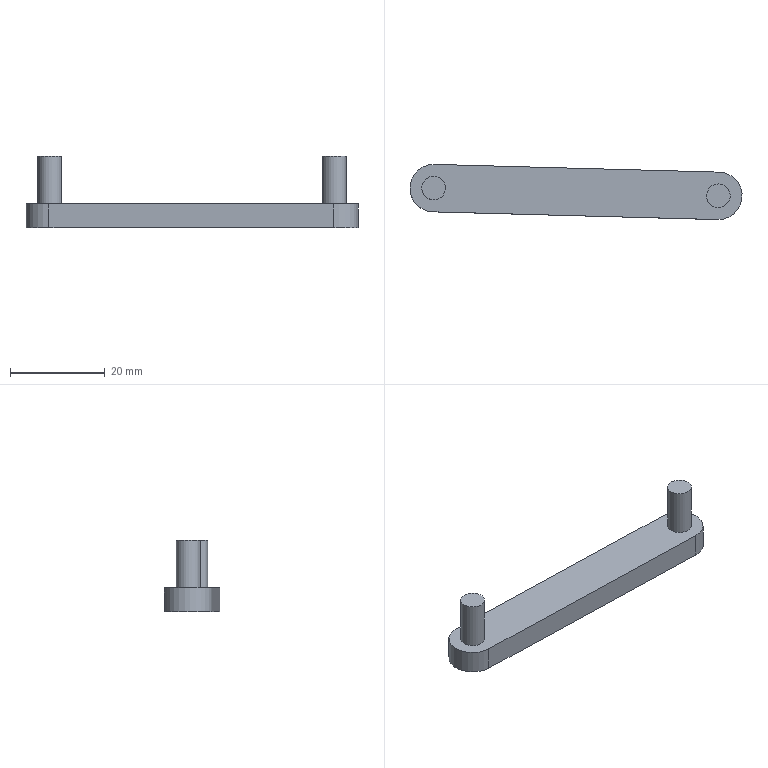Component | NX | CONN_ROD_2 | 1 solid | 10 faces | box 69.98 x 11.63 x 15 mm | volume 3785 mm3 | plane 6 | cylinder 4 | commonest cylinder face diameters 10 x2 5 x2
STEP:
#1=CARTESIAN_POINT('',(0.,0.,0.));
#2=DIRECTION('',(0.,0.,1.));
#3=DIRECTION('',(1.,0.,0.));
#4=AXIS2_PLACEMENT_3D('',#1,#2,#3);
#5=CARTESIAN_POINT('',(-59.864,-73.595,-2.5));
#6=VERTEX_POINT('',#5);
#7=CARTESIAN_POINT('',(-119.842,-71.969,-2.5));
#8=VERTEX_POINT('',#7);
#9=CARTESIAN_POINT('',(-59.864,-73.595,-2.5));
#10=DIRECTION('',(-0.9996,0.0271,0.));
#11=VECTOR('',#10,1.);
#12=LINE('',#9,#11);
#13=CARTESIAN_POINT('',(-59.864,-73.595,2.5));
#14=DIRECTION('',(-0.0271,-0.9996,0.));
#15=DIRECTION('',(0.9996,-0.0271,0.));
#16=AXIS2_PLACEMENT_3D('',#13,#14,#15);
#17=PLANE('',#16);
#18=CARTESIAN_POINT('',(0.,-5.));
#19=DIRECTION('',(-1.,0.));
#20=VECTOR('',#19,1.);
#21=LINE('',#18,#20);
#22=(GEOMETRIC_REPRESENTATION_CONTEXT(2)PARAMETRIC_REPRESENTATION_CONTEXT()REPRESENTATION_CONTEXT('',''));
#23=DEFINITIONAL_REPRESENTATION('',(#21),#22);
#24=PCURVE('',#17,#23);
#25=CARTESIAN_POINT('',(-119.978,-76.967,-2.5));
#26=DIRECTION('',(0.,0.,1.));
#27=DIRECTION('',(-0.0271,-0.9996,0.));
#28=AXIS2_PLACEMENT_3D('',#25,#26,#27);
#29=PLANE('',#28);
#30=CARTESIAN_POINT('',(-5.,60.));
#31=DIRECTION('',(-0.,-1.));
#32=VECTOR('',#31,1.);
#33=LINE('',#30,#32);
#34=(GEOMETRIC_REPRESENTATION_CONTEXT(2)PARAMETRIC_REPRESENTATION_CONTEXT()REPRESENTATION_CONTEXT('',''));
#35=DEFINITIONAL_REPRESENTATION('',(#33),#34);
#36=PCURVE('',#29,#35);
#37=SURFACE_CURVE('',#12,(#24,#36),.PCURVE_S1.);
#38=EDGE_CURVE('',#6,#8,#37,.T.);
#39=ORIENTED_EDGE('',*,*,#38,.T.);
#40=CARTESIAN_POINT('',(-119.842,-71.969,2.5));
#41=VERTEX_POINT('',#40);
#42=CARTESIAN_POINT('',(-119.842,-71.969,2.5));
#43=DIRECTION('',(0.,0.,-1.));
#44=VECTOR('',#43,1.);
#45=LINE('',#42,#44);
#46=CARTESIAN_POINT('',(-60.,0.));
#47=DIRECTION('',(0.,-1.));
#48=VECTOR('',#47,1.);
#49=LINE('',#46,#48);
#50=(GEOMETRIC_REPRESENTATION_CONTEXT(2)PARAMETRIC_REPRESENTATION_CONTEXT()REPRESENTATION_CONTEXT('',''));
#51=DEFINITIONAL_REPRESENTATION('',(#49),#50);
#52=PCURVE('',#17,#51);
#53=CARTESIAN_POINT('',(-119.978,-76.967,2.5));
#54=DIRECTION('',(0.,0.,-1.));
#55=DIRECTION('',(0.0271,0.9996,0.));
#56=AXIS2_PLACEMENT_3D('',#53,#54,#55);
#57=CYLINDRICAL_SURFACE('',#56,5.);
#58=CARTESIAN_POINT('',(6.283,0.));
#59=DIRECTION('',(0.,1.));
#60=VECTOR('',#59,1.);
#61=LINE('',#58,#60);
#62=(GEOMETRIC_REPRESENTATION_CONTEXT(2)PARAMETRIC_REPRESENTATION_CONTEXT()REPRESENTATION_CONTEXT('',''));
#63=DEFINITIONAL_REPRESENTATION('',(#61),#62);
#64=PCURVE('',#57,#63);
#65=SURFACE_CURVE('',#45,(#52,#64),.PCURVE_S1.);
#66=EDGE_CURVE('',#41,#8,#65,.T.);
#67=ORIENTED_EDGE('',*,*,#66,.F.);
#68=CARTESIAN_POINT('',(-59.864,-73.595,2.5));
#69=VERTEX_POINT('',#68);
#70=CARTESIAN_POINT('',(-59.864,-73.595,2.5));
#71=DIRECTION('',(-0.9996,0.0271,0.));
#72=VECTOR('',#71,1.);
#73=LINE('',#70,#72);
#74=CARTESIAN_POINT('',(0.,0.));
#75=DIRECTION('',(-1.,0.));
#76=VECTOR('',#75,1.);
#77=LINE('',#74,#76);
#78=(GEOMETRIC_REPRESENTATION_CONTEXT(2)PARAMETRIC_REPRESENTATION_CONTEXT()REPRESENTATION_CONTEXT('',''));
#79=DEFINITIONAL_REPRESENTATION('',(#77),#78);
#80=PCURVE('',#17,#79);
#81=CARTESIAN_POINT('',(-119.978,-76.967,2.5));
#82=DIRECTION('',(0.,0.,1.));
#83=DIRECTION('',(-0.0271,-0.9996,0.));
#84=AXIS2_PLACEMENT_3D('',#81,#82,#83);
#85=PLANE('',#84);
#86=CARTESIAN_POINT('',(-5.,60.));
#87=DIRECTION('',(-0.,-1.));
#88=VECTOR('',#87,1.);
#89=LINE('',#86,#88);
#90=(GEOMETRIC_REPRESENTATION_CONTEXT(2)PARAMETRIC_REPRESENTATION_CONTEXT()REPRESENTATION_CONTEXT('',''));
#91=DEFINITIONAL_REPRESENTATION('',(#89),#90);
#92=PCURVE('',#85,#91);
#93=SURFACE_CURVE('',#73,(#80,#92),.PCURVE_S1.);
#94=EDGE_CURVE('',#69,#41,#93,.T.);
#95=ORIENTED_EDGE('',*,*,#94,.F.);
#96=CARTESIAN_POINT('',(-59.864,-73.595,2.5));
#97=DIRECTION('',(0.,0.,-1.));
#98=VECTOR('',#97,1.);
#99=LINE('',#96,#98);
#100=CARTESIAN_POINT('',(0.,0.));
#101=DIRECTION('',(0.,-1.));
#102=VECTOR('',#101,1.);
#103=LINE('',#100,#102);
#104=(GEOMETRIC_REPRESENTATION_CONTEXT(2)PARAMETRIC_REPRESENTATION_CONTEXT()REPRESENTATION_CONTEXT('',''));
#105=DEFINITIONAL_REPRESENTATION('',(#103),#104);
#106=PCURVE('',#17,#105);
#107=CARTESIAN_POINT('',(-60.,-78.593,2.5));
#108=DIRECTION('',(0.,0.,-1.));
#109=DIRECTION('',(0.0271,0.9996,0.));
#110=AXIS2_PLACEMENT_3D('',#107,#108,#109);
#111=CYLINDRICAL_SURFACE('',#110,5.);
#112=CARTESIAN_POINT('',(0.,0.));
#113=DIRECTION('',(0.,1.));
#114=VECTOR('',#113,1.);
#115=LINE('',#112,#114);
#116=(GEOMETRIC_REPRESENTATION_CONTEXT(2)PARAMETRIC_REPRESENTATION_CONTEXT()REPRESENTATION_CONTEXT('',''));
#117=DEFINITIONAL_REPRESENTATION('',(#115),#116);
#118=PCURVE('',#111,#117);
#119=SURFACE_CURVE('',#99,(#106,#118),.PCURVE_S1.);
#120=EDGE_CURVE('',#69,#6,#119,.T.);
#121=ORIENTED_EDGE('',*,*,#120,.T.);
#122=EDGE_LOOP('',(#39,#67,#95,#121));
#123=FACE_BOUND('',#122,.T.);
#124=ADVANCED_FACE('',(#123),#17,.F.);
#125=CARTESIAN_POINT('',(-120.113,-81.965,-2.5));
#126=VERTEX_POINT('',#125);
#127=CARTESIAN_POINT('',(-119.978,-76.967,-2.5));
#128=DIRECTION('',(0.,0.,1.));
#129=DIRECTION('',(-0.0271,-0.9996,0.));
#130=AXIS2_PLACEMENT_3D('',#127,#128,#129);
#131=CIRCLE('',#130,5.);
#132=CARTESIAN_POINT('',(9.425,5.));
#133=DIRECTION('',(-1.,0.));
#134=VECTOR('',#133,1.);
#135=LINE('',#132,#134);
#136=(GEOMETRIC_REPRESENTATION_CONTEXT(2)PARAMETRIC_REPRESENTATION_CONTEXT()REPRESENTATION_CONTEXT('',''));
#137=DEFINITIONAL_REPRESENTATION('',(#135),#136);
#138=PCURVE('',#57,#137);
#139=CARTESIAN_POINT('',(0.,0.));
#140=DIRECTION('',(1.,-0.));
#141=AXIS2_PLACEMENT_2D('',#139,#140);
#142=CIRCLE('',#141,5.);
#143=(GEOMETRIC_REPRESENTATION_CONTEXT(2)PARAMETRIC_REPRESENTATION_CONTEXT()REPRESENTATION_CONTEXT('',''));
#144=DEFINITIONAL_REPRESENTATION('',(#142),#143);
#145=PCURVE('',#29,#144);
#146=SURFACE_CURVE('',#131,(#138,#145),.PCURVE_S1.);
#147=EDGE_CURVE('',#8,#126,#146,.T.);
#148=ORIENTED_EDGE('',*,*,#147,.T.);
#149=CARTESIAN_POINT('',(-120.113,-81.965,2.5));
#150=VERTEX_POINT('',#149);
#151=CARTESIAN_POINT('',(-120.113,-81.965,2.5));
#152=DIRECTION('',(0.,0.,-1.));
#153=VECTOR('',#152,1.);
#154=LINE('',#151,#153);
#155=CARTESIAN_POINT('',(3.142,0.));
#156=DIRECTION('',(0.,1.));
#157=VECTOR('',#156,1.);
#158=LINE('',#155,#157);
#159=(GEOMETRIC_REPRESENTATION_CONTEXT(2)PARAMETRIC_REPRESENTATION_CONTEXT()REPRESENTATION_CONTEXT('',''));
#160=DEFINITIONAL_REPRESENTATION('',(#158),#159);
#161=PCURVE('',#57,#160);
#162=CARTESIAN_POINT('',(-120.113,-81.965,2.5));
#163=DIRECTION('',(0.0271,0.9996,0.));
#164=DIRECTION('',(-0.9996,0.0271,0.));
#165=AXIS2_PLACEMENT_3D('',#162,#163,#164);
#166=PLANE('',#165);
#167=CARTESIAN_POINT('',(0.,0.));
#168=DIRECTION('',(0.,-1.));
#169=VECTOR('',#168,1.);
#170=LINE('',#167,#169);
#171=(GEOMETRIC_REPRESENTATION_CONTEXT(2)PARAMETRIC_REPRESENTATION_CONTEXT()REPRESENTATION_CONTEXT('',''));
#172=DEFINITIONAL_REPRESENTATION('',(#170),#171);
#173=PCURVE('',#166,#172);
#174=SURFACE_CURVE('',#154,(#161,#173),.PCURVE_S1.);
#175=EDGE_CURVE('',#150,#126,#174,.T.);
#176=ORIENTED_EDGE('',*,*,#175,.F.);
#177=CARTESIAN_POINT('',(-119.978,-76.967,2.5));
#178=DIRECTION('',(0.,0.,1.));
#179=DIRECTION('',(-0.0271,-0.9996,0.));
#180=AXIS2_PLACEMENT_3D('',#177,#178,#179);
#181=CIRCLE('',#180,5.);
#182=CARTESIAN_POINT('',(9.425,0.));
#183=DIRECTION('',(-1.,0.));
#184=VECTOR('',#183,1.);
#185=LINE('',#182,#184);
#186=(GEOMETRIC_REPRESENTATION_CONTEXT(2)PARAMETRIC_REPRESENTATION_CONTEXT()REPRESENTATION_CONTEXT('',''));
#187=DEFINITIONAL_REPRESENTATION('',(#185),#186);
#188=PCURVE('',#57,#187);
#189=CARTESIAN_POINT('',(0.,0.));
#190=DIRECTION('',(1.,-0.));
#191=AXIS2_PLACEMENT_2D('',#189,#190);
#192=CIRCLE('',#191,5.);
#193=(GEOMETRIC_REPRESENTATION_CONTEXT(2)PARAMETRIC_REPRESENTATION_CONTEXT()REPRESENTATION_CONTEXT('',''));
#194=DEFINITIONAL_REPRESENTATION('',(#192),#193);
#195=PCURVE('',#85,#194);
#196=SURFACE_CURVE('',#181,(#188,#195),.PCURVE_S1.);
#197=EDGE_CURVE('',#41,#150,#196,.T.);
#198=ORIENTED_EDGE('',*,*,#197,.F.);
#199=ORIENTED_EDGE('',*,*,#66,.T.);
#200=EDGE_LOOP('',(#148,#176,#198,#199));
#201=FACE_BOUND('',#200,.T.);
#202=ADVANCED_FACE('',(#201),#57,.T.);
#203=CARTESIAN_POINT('',(-60.136,-83.592,-2.5));
#204=VERTEX_POINT('',#203);
#205=CARTESIAN_POINT('',(-120.113,-81.965,-2.5));
#206=DIRECTION('',(0.9996,-0.0271,0.));
#207=VECTOR('',#206,1.);
#208=LINE('',#205,#207);
#209=CARTESIAN_POINT('',(0.,-5.));
#210=DIRECTION('',(-1.,0.));
#211=VECTOR('',#210,1.);
#212=LINE('',#209,#211);
#213=(GEOMETRIC_REPRESENTATION_CONTEXT(2)PARAMETRIC_REPRESENTATION_CONTEXT()REPRESENTATION_CONTEXT('',''));
#214=DEFINITIONAL_REPRESENTATION('',(#212),#213);
#215=PCURVE('',#166,#214);
#216=CARTESIAN_POINT('',(5.,0.));
#217=DIRECTION('',(0.,1.));
#218=VECTOR('',#217,1.);
#219=LINE('',#216,#218);
#220=(GEOMETRIC_REPRESENTATION_CONTEXT(2)PARAMETRIC_REPRESENTATION_CONTEXT()REPRESENTATION_CONTEXT('',''));
#221=DEFINITIONAL_REPRESENTATION('',(#219),#220);
#222=PCURVE('',#29,#221);
#223=SURFACE_CURVE('',#208,(#215,#222),.PCURVE_S1.);
#224=EDGE_CURVE('',#126,#204,#223,.T.);
#225=ORIENTED_EDGE('',*,*,#224,.T.);
#226=CARTESIAN_POINT('',(-60.136,-83.592,2.5));
#227=VERTEX_POINT('',#226);
#228=CARTESIAN_POINT('',(-60.136,-83.592,2.5));
#229=DIRECTION('',(0.,0.,-1.));
#230=VECTOR('',#229,1.);
#231=LINE('',#228,#230);
#232=CARTESIAN_POINT('',(-60.,0.));
#233=DIRECTION('',(0.,-1.));
#234=VECTOR('',#233,1.);
#235=LINE('',#232,#234);
#236=(GEOMETRIC_REPRESENTATION_CONTEXT(2)PARAMETRIC_REPRESENTATION_CONTEXT()REPRESENTATION_CONTEXT('',''));
#237=DEFINITIONAL_REPRESENTATION('',(#235),#236);
#238=PCURVE('',#166,#237);
#239=CARTESIAN_POINT('',(3.142,0.));
#240=DIRECTION('',(0.,1.));
#241=VECTOR('',#240,1.);
#242=LINE('',#239,#241);
#243=(GEOMETRIC_REPRESENTATION_CONTEXT(2)PARAMETRIC_REPRESENTATION_CONTEXT()REPRESENTATION_CONTEXT('',''));
#244=DEFINITIONAL_REPRESENTATION('',(#242),#243);
#245=PCURVE('',#111,#244);
#246=SURFACE_CURVE('',#231,(#238,#245),.PCURVE_S1.);
#247=EDGE_CURVE('',#227,#204,#246,.T.);
#248=ORIENTED_EDGE('',*,*,#247,.F.);
#249=CARTESIAN_POINT('',(-120.113,-81.965,2.5));
#250=DIRECTION('',(0.9996,-0.0271,0.));
#251=VECTOR('',#250,1.);
#252=LINE('',#249,#251);
#253=CARTESIAN_POINT('',(0.,0.));
#254=DIRECTION('',(-1.,0.));
#255=VECTOR('',#254,1.);
#256=LINE('',#253,#255);
#257=(GEOMETRIC_REPRESENTATION_CONTEXT(2)PARAMETRIC_REPRESENTATION_CONTEXT()REPRESENTATION_CONTEXT('',''));
#258=DEFINITIONAL_REPRESENTATION('',(#256),#257);
#259=PCURVE('',#166,#258);
#260=CARTESIAN_POINT('',(5.,0.));
#261=DIRECTION('',(0.,1.));
#262=VECTOR('',#261,1.);
#263=LINE('',#260,#262);
#264=(GEOMETRIC_REPRESENTATION_CONTEXT(2)PARAMETRIC_REPRESENTATION_CONTEXT()REPRESENTATION_CONTEXT('',''));
#265=DEFINITIONAL_REPRESENTATION('',(#263),#264);
#266=PCURVE('',#85,#265);
#267=SURFACE_CURVE('',#252,(#259,#266),.PCURVE_S1.);
#268=EDGE_CURVE('',#150,#227,#267,.T.);
#269=ORIENTED_EDGE('',*,*,#268,.F.);
#270=ORIENTED_EDGE('',*,*,#175,.T.);
#271=EDGE_LOOP('',(#225,#248,#269,#270));
#272=FACE_BOUND('',#271,.T.);
#273=ADVANCED_FACE('',(#272),#166,.F.);
#274=CARTESIAN_POINT('',(-60.,-78.593,-2.5));
#275=DIRECTION('',(0.,0.,1.));
#276=DIRECTION('',(-0.0271,-0.9996,0.));
#277=AXIS2_PLACEMENT_3D('',#274,#275,#276);
#278=CIRCLE('',#277,5.);
#279=CARTESIAN_POINT('',(3.142,5.));
#280=DIRECTION('',(-1.,0.));
#281=VECTOR('',#280,1.);
#282=LINE('',#279,#281);
#283=(GEOMETRIC_REPRESENTATION_CONTEXT(2)PARAMETRIC_REPRESENTATION_CONTEXT()REPRESENTATION_CONTEXT('',''));
#284=DEFINITIONAL_REPRESENTATION('',(#282),#283);
#285=PCURVE('',#111,#284);
#286=CARTESIAN_POINT('',(0.,60.));
#287=DIRECTION('',(1.,0.));
#288=AXIS2_PLACEMENT_2D('',#286,#287);
#289=CIRCLE('',#288,5.);
#290=(GEOMETRIC_REPRESENTATION_CONTEXT(2)PARAMETRIC_REPRESENTATION_CONTEXT()REPRESENTATION_CONTEXT('',''));
#291=DEFINITIONAL_REPRESENTATION('',(#289),#290);
#292=PCURVE('',#29,#291);
#293=SURFACE_CURVE('',#278,(#285,#292),.PCURVE_S1.);
#294=EDGE_CURVE('',#204,#6,#293,.T.);
#295=ORIENTED_EDGE('',*,*,#294,.T.);
#296=ORIENTED_EDGE('',*,*,#120,.F.);
#297=CARTESIAN_POINT('',(-60.,-78.593,2.5));
#298=DIRECTION('',(0.,0.,1.));
#299=DIRECTION('',(-0.0271,-0.9996,0.));
#300=AXIS2_PLACEMENT_3D('',#297,#298,#299);
#301=CIRCLE('',#300,5.);
#302=CARTESIAN_POINT('',(3.142,0.));
#303=DIRECTION('',(-1.,0.));
#304=VECTOR('',#303,1.);
#305=LINE('',#302,#304);
#306=(GEOMETRIC_REPRESENTATION_CONTEXT(2)PARAMETRIC_REPRESENTATION_CONTEXT()REPRESENTATION_CONTEXT('',''));
#307=DEFINITIONAL_REPRESENTATION('',(#305),#306);
#308=PCURVE('',#111,#307);
#309=CARTESIAN_POINT('',(0.,60.));
#310=DIRECTION('',(1.,0.));
#311=AXIS2_PLACEMENT_2D('',#309,#310);
#312=CIRCLE('',#311,5.);
#313=(GEOMETRIC_REPRESENTATION_CONTEXT(2)PARAMETRIC_REPRESENTATION_CONTEXT()REPRESENTATION_CONTEXT('',''));
#314=DEFINITIONAL_REPRESENTATION('',(#312),#313);
#315=PCURVE('',#85,#314);
#316=SURFACE_CURVE('',#301,(#308,#315),.PCURVE_S1.);
#317=EDGE_CURVE('',#227,#69,#316,.T.);
#318=ORIENTED_EDGE('',*,*,#317,.F.);
#319=ORIENTED_EDGE('',*,*,#247,.T.);
#320=EDGE_LOOP('',(#295,#296,#318,#319));
#321=FACE_BOUND('',#320,.T.);
#322=ADVANCED_FACE('',(#321),#111,.T.);
#323=CARTESIAN_POINT('',(-60.068,-81.092,2.5));
#324=VERTEX_POINT('',#323);
#325=CARTESIAN_POINT('',(-60.,-78.593,2.5));
#326=DIRECTION('',(0.,0.,-1.));
#327=DIRECTION('',(-0.0271,-0.9996,0.));
#328=AXIS2_PLACEMENT_3D('',#325,#326,#327);
#329=CIRCLE('',#328,2.5);
#330=CARTESIAN_POINT('',(2.5,60.));
#331=CARTESIAN_POINT('',(2.5,55.67));
#332=CARTESIAN_POINT('',(-1.25,57.835));
#333=CARTESIAN_POINT('',(-5.,60.));
#334=CARTESIAN_POINT('',(-1.25,62.165));
#335=CARTESIAN_POINT('',(2.5,64.33));
#336=CARTESIAN_POINT('',(2.5,60.));
#337=(BOUNDED_CURVE()B_SPLINE_CURVE(2,(#330,#331,#332,#333,#334,#335,#336),.UNSPECIFIED.,.T.,.F.)B_SPLINE_CURVE_WITH_KNOTS((1,2,2,2,2,1),(-2.094,0.,2.094,4.189,6.283,8.378),.UNSPECIFIED.)CURVE()GEOMETRIC_REPRESENTATION_ITEM()RATIONAL_B_SPLINE_CURVE((1.,0.5,1.,0.5,1.,0.5,1.))REPRESENTATION_ITEM(''));
#338=(GEOMETRIC_REPRESENTATION_CONTEXT(2)PARAMETRIC_REPRESENTATION_CONTEXT()REPRESENTATION_CONTEXT('',''));
#339=DEFINITIONAL_REPRESENTATION('',(#337),#338);
#340=PCURVE('',#85,#339);
#341=CARTESIAN_POINT('',(-60.,-78.593,12.5));
#342=DIRECTION('',(0.,0.,-1.));
#343=DIRECTION('',(0.0271,0.9996,0.));
#344=AXIS2_PLACEMENT_3D('',#341,#342,#343);
#345=CYLINDRICAL_SURFACE('',#344,2.5);
#346=CARTESIAN_POINT('',(3.142,10.));
#347=DIRECTION('',(1.,0.));
#348=VECTOR('',#347,1.);
#349=LINE('',#346,#348);
#350=(GEOMETRIC_REPRESENTATION_CONTEXT(2)PARAMETRIC_REPRESENTATION_CONTEXT()REPRESENTATION_CONTEXT('',''));
#351=DEFINITIONAL_REPRESENTATION('',(#349),#350);
#352=PCURVE('',#345,#351);
#353=SURFACE_CURVE('',#329,(#340,#352),.PCURVE_S1.);
#354=EDGE_CURVE('',#324,#324,#353,.T.);
#355=ORIENTED_EDGE('',*,*,#354,.T.);
#356=EDGE_LOOP('',(#355));
#357=FACE_BOUND('',#356,.T.);
#358=CARTESIAN_POINT('',(-120.046,-79.466,2.5));
#359=VERTEX_POINT('',#358);
#360=CARTESIAN_POINT('',(-119.978,-76.967,2.5));
#361=DIRECTION('',(0.,0.,-1.));
#362=DIRECTION('',(-0.0271,-0.9996,0.));
#363=AXIS2_PLACEMENT_3D('',#360,#361,#362);
#364=CIRCLE('',#363,2.5);
#365=CARTESIAN_POINT('',(2.5,0.));
#366=CARTESIAN_POINT('',(2.5,-4.33));
#367=CARTESIAN_POINT('',(-1.25,-2.165));
#368=CARTESIAN_POINT('',(-5.,-0.));
#369=CARTESIAN_POINT('',(-1.25,2.165));
#370=CARTESIAN_POINT('',(2.5,4.33));
#371=CARTESIAN_POINT('',(2.5,0.));
#372=(BOUNDED_CURVE()B_SPLINE_CURVE(2,(#365,#366,#367,#368,#369,#370,#371),.UNSPECIFIED.,.T.,.F.)B_SPLINE_CURVE_WITH_KNOTS((1,2,2,2,2,1),(-2.094,0.,2.094,4.189,6.283,8.378),.UNSPECIFIED.)CURVE()GEOMETRIC_REPRESENTATION_ITEM()RATIONAL_B_SPLINE_CURVE((1.,0.5,1.,0.5,1.,0.5,1.))REPRESENTATION_ITEM(''));
#373=(GEOMETRIC_REPRESENTATION_CONTEXT(2)PARAMETRIC_REPRESENTATION_CONTEXT()REPRESENTATION_CONTEXT('',''));
#374=DEFINITIONAL_REPRESENTATION('',(#372),#373);
#375=PCURVE('',#85,#374);
#376=CARTESIAN_POINT('',(-119.978,-76.967,12.5));
#377=DIRECTION('',(0.,0.,-1.));
#378=DIRECTION('',(0.0271,0.9996,0.));
#379=AXIS2_PLACEMENT_3D('',#376,#377,#378);
#380=CYLINDRICAL_SURFACE('',#379,2.5);
#381=CARTESIAN_POINT('',(3.142,10.));
#382=DIRECTION('',(1.,0.));
#383=VECTOR('',#382,1.);
#384=LINE('',#381,#383);
#385=(GEOMETRIC_REPRESENTATION_CONTEXT(2)PARAMETRIC_REPRESENTATION_CONTEXT()REPRESENTATION_CONTEXT('',''));
#386=DEFINITIONAL_REPRESENTATION('',(#384),#385);
#387=PCURVE('',#380,#386);
#388=SURFACE_CURVE('',#364,(#375,#387),.PCURVE_S1.);
#389=EDGE_CURVE('',#359,#359,#388,.T.);
#390=ORIENTED_EDGE('',*,*,#389,.T.);
#391=EDGE_LOOP('',(#390));
#392=FACE_BOUND('',#391,.T.);
#393=ORIENTED_EDGE('',*,*,#94,.T.);
#394=ORIENTED_EDGE('',*,*,#197,.T.);
#395=ORIENTED_EDGE('',*,*,#268,.T.);
#396=ORIENTED_EDGE('',*,*,#317,.T.);
#397=EDGE_LOOP('',(#393,#394,#395,#396));
#398=FACE_BOUND('',#397,.T.);
#399=ADVANCED_FACE('',(#357,#392,#398),#85,.T.);
#400=ORIENTED_EDGE('',*,*,#38,.F.);
#401=ORIENTED_EDGE('',*,*,#294,.F.);
#402=ORIENTED_EDGE('',*,*,#224,.F.);
#403=ORIENTED_EDGE('',*,*,#147,.F.);
#404=EDGE_LOOP('',(#400,#401,#402,#403));
#405=FACE_BOUND('',#404,.T.);
#406=ADVANCED_FACE('',(#405),#29,.F.);
#407=CARTESIAN_POINT('',(-120.046,-79.466,12.5));
#408=VERTEX_POINT('',#407);
#409=CARTESIAN_POINT('',(-119.978,-76.967,12.5));
#410=DIRECTION('',(0.,0.,-1.));
#411=DIRECTION('',(-0.0271,-0.9996,0.));
#412=AXIS2_PLACEMENT_3D('',#409,#410,#411);
#413=CIRCLE('',#412,2.5);
#414=CARTESIAN_POINT('',(3.142,0.));
#415=DIRECTION('',(1.,0.));
#416=VECTOR('',#415,1.);
#417=LINE('',#414,#416);
#418=(GEOMETRIC_REPRESENTATION_CONTEXT(2)PARAMETRIC_REPRESENTATION_CONTEXT()REPRESENTATION_CONTEXT('',''));
#419=DEFINITIONAL_REPRESENTATION('',(#417),#418);
#420=PCURVE('',#380,#419);
#421=CARTESIAN_POINT('',(-119.978,-76.967,12.5));
#422=DIRECTION('',(0.,0.,-1.));
#423=DIRECTION('',(0.0271,0.9996,0.));
#424=AXIS2_PLACEMENT_3D('',#421,#422,#423);
#425=PLANE('',#424);
#426=CARTESIAN_POINT('',(0.,0.));
#427=DIRECTION('',(-1.,0.));
#428=AXIS2_PLACEMENT_2D('',#426,#427);
#429=CIRCLE('',#428,2.5);
#430=(GEOMETRIC_REPRESENTATION_CONTEXT(2)PARAMETRIC_REPRESENTATION_CONTEXT()REPRESENTATION_CONTEXT('',''));
#431=DEFINITIONAL_REPRESENTATION('',(#429),#430);
#432=PCURVE('',#425,#431);
#433=SURFACE_CURVE('',#413,(#420,#432),.PCURVE_S1.);
#434=EDGE_CURVE('',#408,#408,#433,.T.);
#435=ORIENTED_EDGE('',*,*,#434,.T.);
#436=CARTESIAN_POINT('',(-120.046,-79.466,12.5));
#437=CARTESIAN_POINT('',(-120.046,-79.466,2.5));
#438=B_SPLINE_CURVE_WITH_KNOTS('',1,(#436,#437),.UNSPECIFIED.,.F.,.F.,(2,2),(0.,10.),.PIECEWISE_BEZIER_KNOTS.);
#439=CARTESIAN_POINT('',(9.425,0.));
#440=DIRECTION('',(0.,1.));
#441=VECTOR('',#440,1.);
#442=LINE('',#439,#441);
#443=(GEOMETRIC_REPRESENTATION_CONTEXT(2)PARAMETRIC_REPRESENTATION_CONTEXT()REPRESENTATION_CONTEXT('',''));
#444=DEFINITIONAL_REPRESENTATION('',(#442),#443);
#445=PCURVE('',#380,#444);
#446=CARTESIAN_POINT('',(3.142,0.));
#447=DIRECTION('',(0.,1.));
#448=VECTOR('',#447,1.);
#449=LINE('',#446,#448);
#450=(GEOMETRIC_REPRESENTATION_CONTEXT(2)PARAMETRIC_REPRESENTATION_CONTEXT()REPRESENTATION_CONTEXT('',''));
#451=DEFINITIONAL_REPRESENTATION('',(#449),#450);
#452=PCURVE('',#380,#451);
#453=SEAM_CURVE('',#438,(#445,#452),.PCURVE_S1.);
#454=EDGE_CURVE('',#408,#359,#453,.T.);
#455=ORIENTED_EDGE('',*,*,#454,.T.);
#456=ORIENTED_EDGE('',*,*,#389,.F.);
#457=ORIENTED_EDGE('',*,*,#454,.F.);
#458=EDGE_LOOP('',(#435,#455,#456,#457));
#459=FACE_BOUND('',#458,.T.);
#460=ADVANCED_FACE('',(#459),#380,.T.);
#461=ORIENTED_EDGE('',*,*,#434,.F.);
#462=EDGE_LOOP('',(#461));
#463=FACE_BOUND('',#462,.T.);
#464=ADVANCED_FACE('',(#463),#425,.F.);
#465=CARTESIAN_POINT('',(-60.068,-81.092,12.5));
#466=VERTEX_POINT('',#465);
#467=CARTESIAN_POINT('',(-60.,-78.593,12.5));
#468=DIRECTION('',(0.,0.,-1.));
#469=DIRECTION('',(-0.0271,-0.9996,0.));
#470=AXIS2_PLACEMENT_3D('',#467,#468,#469);
#471=CIRCLE('',#470,2.5);
#472=CARTESIAN_POINT('',(3.142,0.));
#473=DIRECTION('',(1.,0.));
#474=VECTOR('',#473,1.);
#475=LINE('',#472,#474);
#476=(GEOMETRIC_REPRESENTATION_CONTEXT(2)PARAMETRIC_REPRESENTATION_CONTEXT()REPRESENTATION_CONTEXT('',''));
#477=DEFINITIONAL_REPRESENTATION('',(#475),#476);
#478=PCURVE('',#345,#477);
#479=CARTESIAN_POINT('',(-60.,-78.593,12.5));
#480=DIRECTION('',(0.,0.,-1.));
#481=DIRECTION('',(0.0271,0.9996,0.));
#482=AXIS2_PLACEMENT_3D('',#479,#480,#481);
#483=PLANE('',#482);
#484=CARTESIAN_POINT('',(0.,0.));
#485=DIRECTION('',(-1.,-0.));
#486=AXIS2_PLACEMENT_2D('',#484,#485);
#487=CIRCLE('',#486,2.5);
#488=(GEOMETRIC_REPRESENTATION_CONTEXT(2)PARAMETRIC_REPRESENTATION_CONTEXT()REPRESENTATION_CONTEXT('',''));
#489=DEFINITIONAL_REPRESENTATION('',(#487),#488);
#490=PCURVE('',#483,#489);
#491=SURFACE_CURVE('',#471,(#478,#490),.PCURVE_S1.);
#492=EDGE_CURVE('',#466,#466,#491,.T.);
#493=ORIENTED_EDGE('',*,*,#492,.T.);
#494=CARTESIAN_POINT('',(-60.068,-81.092,12.5));
#495=CARTESIAN_POINT('',(-60.068,-81.092,2.5));
#496=B_SPLINE_CURVE_WITH_KNOTS('',1,(#494,#495),.UNSPECIFIED.,.F.,.F.,(2,2),(0.,10.),.PIECEWISE_BEZIER_KNOTS.);
#497=CARTESIAN_POINT('',(9.425,0.));
#498=DIRECTION('',(0.,1.));
#499=VECTOR('',#498,1.);
#500=LINE('',#497,#499);
#501=(GEOMETRIC_REPRESENTATION_CONTEXT(2)PARAMETRIC_REPRESENTATION_CONTEXT()REPRESENTATION_CONTEXT('',''));
#502=DEFINITIONAL_REPRESENTATION('',(#500),#501);
#503=PCURVE('',#345,#502);
#504=CARTESIAN_POINT('',(3.142,0.));
#505=DIRECTION('',(0.,1.));
#506=VECTOR('',#505,1.);
#507=LINE('',#504,#506);
#508=(GEOMETRIC_REPRESENTATION_CONTEXT(2)PARAMETRIC_REPRESENTATION_CONTEXT()REPRESENTATION_CONTEXT('',''));
#509=DEFINITIONAL_REPRESENTATION('',(#507),#508);
#510=PCURVE('',#345,#509);
#511=SEAM_CURVE('',#496,(#503,#510),.PCURVE_S1.);
#512=EDGE_CURVE('',#466,#324,#511,.T.);
#513=ORIENTED_EDGE('',*,*,#512,.T.);
#514=ORIENTED_EDGE('',*,*,#354,.F.);
#515=ORIENTED_EDGE('',*,*,#512,.F.);
#516=EDGE_LOOP('',(#493,#513,#514,#515));
#517=FACE_BOUND('',#516,.T.);
#518=ADVANCED_FACE('',(#517),#345,.T.);
#519=ORIENTED_EDGE('',*,*,#492,.F.);
#520=EDGE_LOOP('',(#519));
#521=FACE_BOUND('',#520,.T.);
#522=ADVANCED_FACE('',(#521),#483,.F.);
#523=CLOSED_SHELL('',(#124,#202,#273,#322,#399,#406,#460,#464,#518,#522));
#524=MANIFOLD_SOLID_BREP('',#523);
#525=(LENGTH_UNIT()NAMED_UNIT(*)SI_UNIT(.MILLI.,.METRE.));
#526=UNCERTAINTY_MEASURE_WITH_UNIT(LENGTH_MEASURE(0.000002),#525,'','');
#527=(NAMED_UNIT(*)PLANE_ANGLE_UNIT()SI_UNIT($,.RADIAN.));
#528=(NAMED_UNIT(*)SI_UNIT($,.STERADIAN.)SOLID_ANGLE_UNIT());
#529=(GEOMETRIC_REPRESENTATION_CONTEXT(3)GLOBAL_UNCERTAINTY_ASSIGNED_CONTEXT((#526))GLOBAL_UNIT_ASSIGNED_CONTEXT((#525,#527,#528))REPRESENTATION_CONTEXT('',''));
#530=ADVANCED_BREP_SHAPE_REPRESENTATION('',(#4,#524),#529);